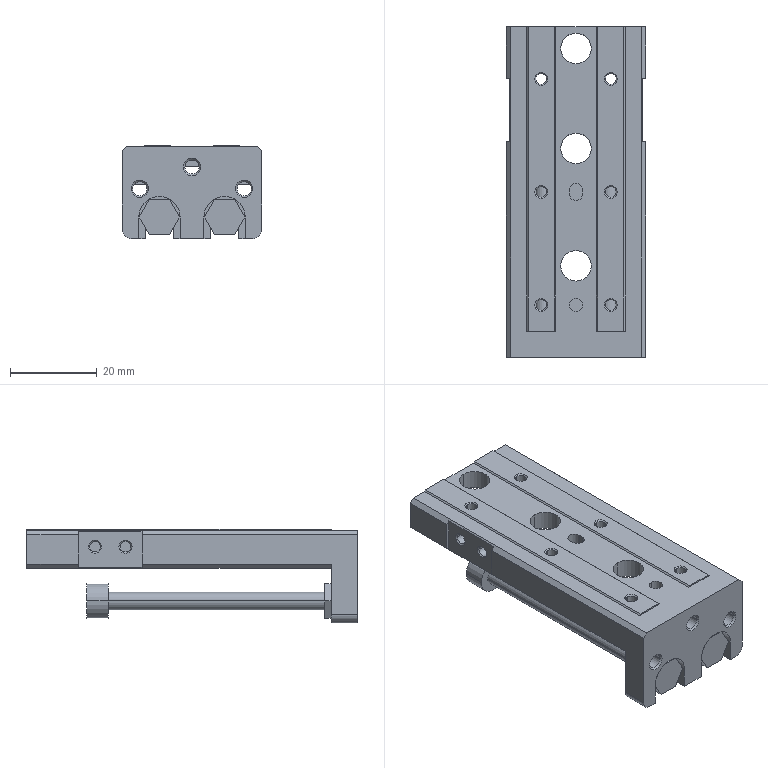Component | SolidWorks | MXQ8-30B-M9N_0_0_MXQ8-30B-M9N_0_0-2_MXQ8-30B-M9N_0_0_2_26-1 | 1 solid | 176 faces | volume 18277 mm3 | plane 93 | cylinder 57 | cone 26 | commonest cylinder face diameters 2.459 x20 7 x6 3.242 x6 4 x6 3 x5 5.7 x4 8 x4 9.5 x2